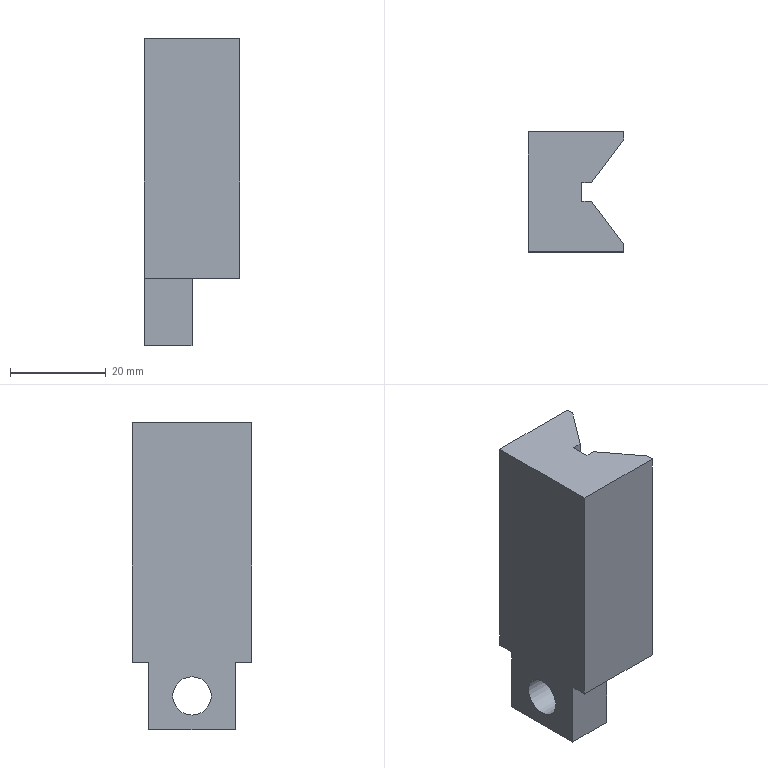Component | NX | V_BLOCK | 1 solid | 17 faces | volume 22209 mm3 | plane 16 | cylinder 1 | commonest cylinder face diameters 8 x1